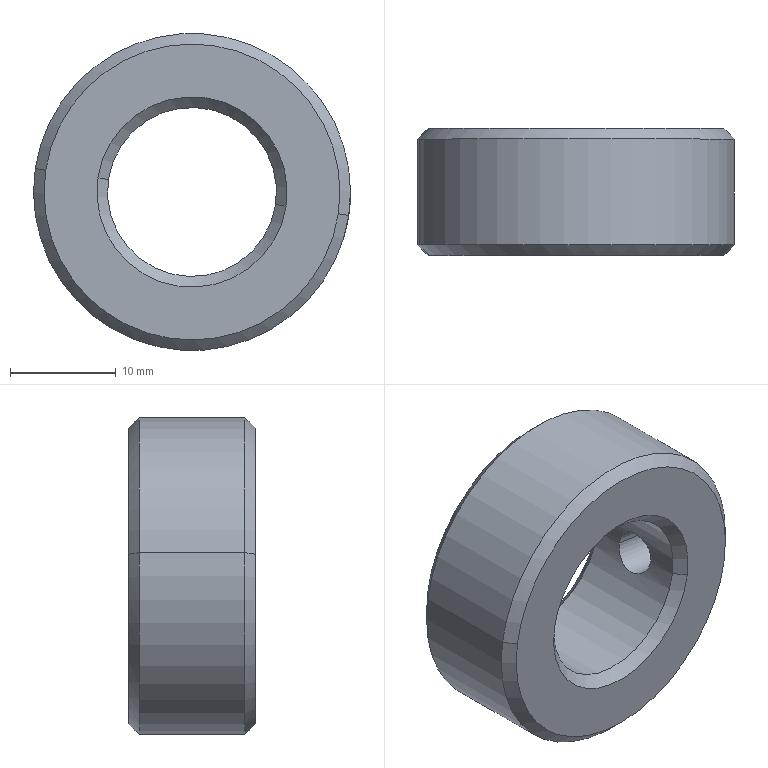Component | SolidWorks | LocatingRing-3 | 1 solid | 16 faces | box 30 x 12 x 30 mm | volume 5828 mm3 | cone 8 | cylinder 6 | plane 2 | commonest cylinder face diameters 30 x2 4.2 x2 16 x2
STEP:
#1=COLOUR_RGB('',0.7922,0.8196,0.9333);
#2=FILL_AREA_STYLE_COLOUR('',#1);
#3=FILL_AREA_STYLE('',(#2));
#4=SURFACE_STYLE_FILL_AREA(#3);
#5=SURFACE_SIDE_STYLE('',(#4));
#6=SURFACE_STYLE_USAGE(.BOTH.,#5);
#7=PRESENTATION_STYLE_ASSIGNMENT((#6));
#8=CARTESIAN_POINT('',(6.686,5.472,-5.796));
#9=VERTEX_POINT('',#8);
#10=CARTESIAN_POINT('',(5.518,5.472,-5.622));
#11=VERTEX_POINT('',#10);
#12=CARTESIAN_POINT('',(6.102,5.472,-5.709));
#13=DIRECTION('',(0.,-1.,0.));
#14=DIRECTION('',(0.9891,0.,-0.1473));
#15=AXIS2_PLACEMENT_3D('',#12,#13,#14);
#16=CIRCLE('',#15,0.5906);
#17=EDGE_CURVE('',#9,#11,#16,.T.);
#18=ORIENTED_EDGE('',*,*,#17,.T.);
#19=CARTESIAN_POINT('',(5.518,5.079,-5.622));
#20=VERTEX_POINT('',#19);
#21=CARTESIAN_POINT('',(5.518,5.512,-5.622));
#22=DIRECTION('',(0.,-1.,0.));
#23=VECTOR('',#22,39.37);
#24=LINE('',#21,#23);
#25=EDGE_CURVE('',#11,#20,#24,.T.);
#26=ORIENTED_EDGE('',*,*,#25,.T.);
#27=CARTESIAN_POINT('',(6.686,5.079,-5.796));
#28=VERTEX_POINT('',#27);
#29=CARTESIAN_POINT('',(6.102,5.079,-5.709));
#30=DIRECTION('',(-0.,1.,-0.));
#31=DIRECTION('',(0.9891,0.,-0.1473));
#32=AXIS2_PLACEMENT_3D('',#29,#30,#31);
#33=CIRCLE('',#32,0.5906);
#34=EDGE_CURVE('',#20,#28,#33,.T.);
#35=ORIENTED_EDGE('',*,*,#34,.T.);
#36=CARTESIAN_POINT('',(6.686,5.193,-5.796));
#37=VERTEX_POINT('',#36);
#38=CARTESIAN_POINT('',(6.686,5.512,-5.796));
#39=DIRECTION('',(0.,-1.,0.));
#40=VECTOR('',#39,39.37);
#41=LINE('',#38,#40);
#42=EDGE_CURVE('',#37,#28,#41,.T.);
#43=ORIENTED_EDGE('',*,*,#42,.F.);
#44=CARTESIAN_POINT('',(6.686,5.358,-5.796));
#45=VERTEX_POINT('',#44);
#46=CARTESIAN_POINT('',(6.686,5.193,-5.796));
#47=CARTESIAN_POINT('',(6.687,5.193,-5.79));
#48=CARTESIAN_POINT('',(6.688,5.193,-5.785));
#49=CARTESIAN_POINT('',(6.689,5.196,-5.774));
#50=CARTESIAN_POINT('',(6.69,5.197,-5.769));
#51=CARTESIAN_POINT('',(6.691,5.201,-5.759));
#52=CARTESIAN_POINT('',(6.691,5.204,-5.754));
#53=CARTESIAN_POINT('',(6.692,5.21,-5.745));
#54=CARTESIAN_POINT('',(6.692,5.213,-5.741));
#55=CARTESIAN_POINT('',(6.693,5.225,-5.73));
#56=CARTESIAN_POINT('',(6.693,5.234,-5.724));
#57=CARTESIAN_POINT('',(6.693,5.254,-5.715));
#58=CARTESIAN_POINT('',(6.693,5.265,-5.713));
#59=CARTESIAN_POINT('',(6.693,5.281,-5.713));
#60=CARTESIAN_POINT('',(6.693,5.286,-5.714));
#61=CARTESIAN_POINT('',(6.693,5.297,-5.716));
#62=CARTESIAN_POINT('',(6.693,5.302,-5.717));
#63=CARTESIAN_POINT('',(6.693,5.312,-5.721));
#64=CARTESIAN_POINT('',(6.693,5.317,-5.724));
#65=CARTESIAN_POINT('',(6.693,5.326,-5.73));
#66=CARTESIAN_POINT('',(6.692,5.33,-5.733));
#67=CARTESIAN_POINT('',(6.692,5.338,-5.741));
#68=CARTESIAN_POINT('',(6.692,5.341,-5.745));
#69=CARTESIAN_POINT('',(6.691,5.347,-5.754));
#70=CARTESIAN_POINT('',(6.691,5.35,-5.759));
#71=CARTESIAN_POINT('',(6.69,5.354,-5.769));
#72=CARTESIAN_POINT('',(6.689,5.356,-5.774));
#73=CARTESIAN_POINT('',(6.688,5.358,-5.785));
#74=CARTESIAN_POINT('',(6.687,5.358,-5.79));
#75=CARTESIAN_POINT('',(6.686,5.358,-5.796));
#76=B_SPLINE_CURVE_WITH_KNOTS('',3,(#46,#47,#48,#49,#50,#51,#52,#53,#54,#55,#56,#57,#58,#59,#60,#61,#62,#63,#64,#65,#66,#67,#68,#69,#70,#71,#72,#73,#74,#75),.UNSPECIFIED.,.F.,.F.,(4,2,2,2,2,2,2,2,2,2,2,2,2,2,4),(0.006572,0.006983,0.007394,0.007804,0.008215,0.009037,0.009858,0.01027,0.01068,0.01109,0.0115,0.01191,0.01232,0.01273,0.01314),.UNSPECIFIED.);
#77=EDGE_CURVE('',#37,#45,#76,.T.);
#78=ORIENTED_EDGE('',*,*,#77,.T.);
#79=CARTESIAN_POINT('',(6.686,5.512,-5.796));
#80=DIRECTION('',(0.,-1.,0.));
#81=VECTOR('',#80,39.37);
#82=LINE('',#79,#81);
#83=EDGE_CURVE('',#9,#45,#82,.T.);
#84=ORIENTED_EDGE('',*,*,#83,.F.);
#85=EDGE_LOOP('',(#18,#26,#35,#43,#78,#84));
#86=FACE_OUTER_BOUND('',#85,.T.);
#87=CARTESIAN_POINT('',(6.102,5.512,-5.709));
#88=DIRECTION('',(0.,-1.,0.));
#89=DIRECTION('',(0.9891,0.,-0.1473));
#90=AXIS2_PLACEMENT_3D('',#87,#88,#89);
#91=CYLINDRICAL_SURFACE('',#90,0.5906);
#92=ADVANCED_FACE('',(#86),#91,.T.);
#93=CARTESIAN_POINT('',(5.557,5.039,-5.627));
#94=VERTEX_POINT('',#93);
#95=CARTESIAN_POINT('',(6.648,5.039,-5.79));
#96=VERTEX_POINT('',#95);
#97=CARTESIAN_POINT('',(6.102,5.039,-5.709));
#98=DIRECTION('',(-0.,1.,-0.));
#99=DIRECTION('',(-0.9891,0.,0.1473));
#100=AXIS2_PLACEMENT_3D('',#97,#98,#99);
#101=CIRCLE('',#100,0.5512);
#102=EDGE_CURVE('',#94,#96,#101,.T.);
#103=ORIENTED_EDGE('',*,*,#102,.T.);
#104=CARTESIAN_POINT('',(6.686,5.079,-5.796));
#105=DIRECTION('',(0.6994,0.7071,-0.1041));
#106=VECTOR('',#105,39.37);
#107=LINE('',#104,#106);
#108=EDGE_CURVE('',#96,#28,#107,.T.);
#109=ORIENTED_EDGE('',*,*,#108,.T.);
#110=ORIENTED_EDGE('',*,*,#34,.F.);
#111=CARTESIAN_POINT('',(5.518,5.079,-5.622));
#112=DIRECTION('',(-0.6994,0.7071,0.1041));
#113=VECTOR('',#112,39.37);
#114=LINE('',#111,#113);
#115=EDGE_CURVE('',#94,#20,#114,.T.);
#116=ORIENTED_EDGE('',*,*,#115,.F.);
#117=EDGE_LOOP('',(#103,#109,#110,#116));
#118=FACE_OUTER_BOUND('',#117,.T.);
#119=CARTESIAN_POINT('',(6.102,5.079,-5.709));
#120=DIRECTION('',(-0.,1.,-0.));
#121=DIRECTION('',(-0.9891,0.,0.1473));
#122=AXIS2_PLACEMENT_3D('',#119,#120,#121);
#123=CONICAL_SURFACE('',#122,0.5906,0.7854);
#124=ADVANCED_FACE('',(#118),#123,.T.);
#125=CARTESIAN_POINT('',(6.414,5.193,-5.755));
#126=VERTEX_POINT('',#125);
#127=CARTESIAN_POINT('',(6.414,5.358,-5.755));
#128=VERTEX_POINT('',#127);
#129=CARTESIAN_POINT('',(6.414,5.193,-5.755));
#130=CARTESIAN_POINT('',(6.413,5.193,-5.76));
#131=CARTESIAN_POINT('',(6.412,5.193,-5.766));
#132=CARTESIAN_POINT('',(6.41,5.196,-5.776));
#133=CARTESIAN_POINT('',(6.409,5.197,-5.781));
#134=CARTESIAN_POINT('',(6.406,5.201,-5.791));
#135=CARTESIAN_POINT('',(6.405,5.204,-5.796));
#136=CARTESIAN_POINT('',(6.402,5.21,-5.804));
#137=CARTESIAN_POINT('',(6.401,5.213,-5.808));
#138=CARTESIAN_POINT('',(6.397,5.225,-5.819));
#139=CARTESIAN_POINT('',(6.395,5.234,-5.825));
#140=CARTESIAN_POINT('',(6.393,5.249,-5.831));
#141=CARTESIAN_POINT('',(6.392,5.254,-5.833));
#142=CARTESIAN_POINT('',(6.391,5.265,-5.835));
#143=CARTESIAN_POINT('',(6.391,5.27,-5.835));
#144=CARTESIAN_POINT('',(6.391,5.281,-5.835));
#145=CARTESIAN_POINT('',(6.391,5.286,-5.835));
#146=CARTESIAN_POINT('',(6.392,5.297,-5.833));
#147=CARTESIAN_POINT('',(6.393,5.302,-5.831));
#148=CARTESIAN_POINT('',(6.395,5.317,-5.825));
#149=CARTESIAN_POINT('',(6.397,5.326,-5.819));
#150=CARTESIAN_POINT('',(6.401,5.338,-5.808));
#151=CARTESIAN_POINT('',(6.402,5.341,-5.804));
#152=CARTESIAN_POINT('',(6.405,5.347,-5.796));
#153=CARTESIAN_POINT('',(6.406,5.35,-5.791));
#154=CARTESIAN_POINT('',(6.409,5.354,-5.781));
#155=CARTESIAN_POINT('',(6.41,5.356,-5.776));
#156=CARTESIAN_POINT('',(6.412,5.358,-5.766));
#157=CARTESIAN_POINT('',(6.413,5.358,-5.76));
#158=CARTESIAN_POINT('',(6.414,5.358,-5.755));
#159=B_SPLINE_CURVE_WITH_KNOTS('',3,(#129,#130,#131,#132,#133,#134,#135,#136,#137,#138,#139,#140,#141,#142,#143,#144,#145,#146,#147,#148,#149,#150,#151,#152,#153,#154,#155,#156,#157,#158),.UNSPECIFIED.,.F.,.F.,(4,2,2,2,2,2,2,2,2,2,2,2,2,2,4),(0.,0.000412,0.0008241,0.001236,0.001648,0.002472,0.002884,0.003296,0.003708,0.00412,0.004944,0.005356,0.005768,0.00618,0.006592),.UNSPECIFIED.);
#160=EDGE_CURVE('',#126,#128,#159,.T.);
#161=ORIENTED_EDGE('',*,*,#160,.F.);
#162=CARTESIAN_POINT('',(6.686,5.193,-5.796));
#163=DIRECTION('',(0.9891,0.,-0.1473));
#164=VECTOR('',#163,39.37);
#165=LINE('',#162,#164);
#166=EDGE_CURVE('',#126,#37,#165,.T.);
#167=ORIENTED_EDGE('',*,*,#166,.T.);
#168=CARTESIAN_POINT('',(6.686,5.358,-5.796));
#169=CARTESIAN_POINT('',(6.686,5.358,-5.801));
#170=CARTESIAN_POINT('',(6.685,5.358,-5.806));
#171=CARTESIAN_POINT('',(6.683,5.356,-5.817));
#172=CARTESIAN_POINT('',(6.682,5.354,-5.822));
#173=CARTESIAN_POINT('',(6.68,5.35,-5.832));
#174=CARTESIAN_POINT('',(6.679,5.347,-5.836));
#175=CARTESIAN_POINT('',(6.677,5.341,-5.845));
#176=CARTESIAN_POINT('',(6.676,5.338,-5.849));
#177=CARTESIAN_POINT('',(6.673,5.326,-5.86));
#178=CARTESIAN_POINT('',(6.671,5.317,-5.866));
#179=CARTESIAN_POINT('',(6.669,5.297,-5.874));
#180=CARTESIAN_POINT('',(6.669,5.286,-5.877));
#181=CARTESIAN_POINT('',(6.669,5.27,-5.877));
#182=CARTESIAN_POINT('',(6.669,5.265,-5.876));
#183=CARTESIAN_POINT('',(6.669,5.254,-5.874));
#184=CARTESIAN_POINT('',(6.67,5.249,-5.872));
#185=CARTESIAN_POINT('',(6.671,5.239,-5.868));
#186=CARTESIAN_POINT('',(6.672,5.234,-5.866));
#187=CARTESIAN_POINT('',(6.673,5.225,-5.86));
#188=CARTESIAN_POINT('',(6.674,5.221,-5.857));
#189=CARTESIAN_POINT('',(6.676,5.213,-5.849));
#190=CARTESIAN_POINT('',(6.677,5.21,-5.845));
#191=CARTESIAN_POINT('',(6.679,5.204,-5.837));
#192=CARTESIAN_POINT('',(6.68,5.201,-5.832));
#193=CARTESIAN_POINT('',(6.682,5.197,-5.822));
#194=CARTESIAN_POINT('',(6.683,5.196,-5.817));
#195=CARTESIAN_POINT('',(6.685,5.193,-5.806));
#196=CARTESIAN_POINT('',(6.686,5.193,-5.801));
#197=CARTESIAN_POINT('',(6.686,5.193,-5.796));
#198=B_SPLINE_CURVE_WITH_KNOTS('',3,(#168,#169,#170,#171,#172,#173,#174,#175,#176,#177,#178,#179,#180,#181,#182,#183,#184,#185,#186,#187,#188,#189,#190,#191,#192,#193,#194,#195,#196,#197),.UNSPECIFIED.,.F.,.F.,(4,2,2,2,2,2,2,2,2,2,2,2,2,2,4),(0.,0.0004108,0.0008215,0.001232,0.001643,0.002465,0.003286,0.003697,0.004108,0.004518,0.004929,0.00534,0.005751,0.006161,0.006572),.UNSPECIFIED.);
#199=EDGE_CURVE('',#45,#37,#198,.T.);
#200=ORIENTED_EDGE('',*,*,#199,.F.);
#201=CARTESIAN_POINT('',(6.686,5.358,-5.796));
#202=DIRECTION('',(0.9891,0.,-0.1473));
#203=VECTOR('',#202,39.37);
#204=LINE('',#201,#203);
#205=EDGE_CURVE('',#128,#45,#204,.T.);
#206=ORIENTED_EDGE('',*,*,#205,.F.);
#207=EDGE_LOOP('',(#161,#167,#200,#206));
#208=FACE_OUTER_BOUND('',#207,.T.);
#209=CARTESIAN_POINT('',(6.686,5.276,-5.796));
#210=DIRECTION('',(0.9891,0.,-0.1473));
#211=DIRECTION('',(0.,1.,0.));
#212=AXIS2_PLACEMENT_3D('',#209,#210,#211);
#213=CYLINDRICAL_SURFACE('',#212,0.08268);
#214=ADVANCED_FACE('',(#208),#213,.F.);
#215=CARTESIAN_POINT('',(6.648,5.512,-5.79));
#216=VERTEX_POINT('',#215);
#217=CARTESIAN_POINT('',(5.557,5.512,-5.627));
#218=VERTEX_POINT('',#217);
#219=CARTESIAN_POINT('',(6.102,5.512,-5.709));
#220=DIRECTION('',(0.,-1.,0.));
#221=DIRECTION('',(0.9891,0.,-0.1473));
#222=AXIS2_PLACEMENT_3D('',#219,#220,#221);
#223=CIRCLE('',#222,0.5512);
#224=EDGE_CURVE('',#216,#218,#223,.T.);
#225=ORIENTED_EDGE('',*,*,#224,.T.);
#226=CARTESIAN_POINT('',(5.518,5.472,-5.622));
#227=DIRECTION('',(-0.6994,-0.7071,0.1041));
#228=VECTOR('',#227,39.37);
#229=LINE('',#226,#228);
#230=EDGE_CURVE('',#218,#11,#229,.T.);
#231=ORIENTED_EDGE('',*,*,#230,.T.);
#232=ORIENTED_EDGE('',*,*,#17,.F.);
#233=CARTESIAN_POINT('',(6.686,5.472,-5.796));
#234=DIRECTION('',(0.6994,-0.7071,-0.1041));
#235=VECTOR('',#234,39.37);
#236=LINE('',#233,#235);
#237=EDGE_CURVE('',#216,#9,#236,.T.);
#238=ORIENTED_EDGE('',*,*,#237,.F.);
#239=EDGE_LOOP('',(#225,#231,#232,#238));
#240=FACE_OUTER_BOUND('',#239,.T.);
#241=CARTESIAN_POINT('',(6.102,5.472,-5.709));
#242=DIRECTION('',(0.,-1.,0.));
#243=DIRECTION('',(0.9891,0.,-0.1473));
#244=AXIS2_PLACEMENT_3D('',#241,#242,#243);
#245=CONICAL_SURFACE('',#244,0.5906,0.7854);
#246=ADVANCED_FACE('',(#240),#245,.T.);
#247=CARTESIAN_POINT('',(6.414,5.079,-5.755));
#248=VERTEX_POINT('',#247);
#249=CARTESIAN_POINT('',(5.791,5.079,-5.662));
#250=VERTEX_POINT('',#249);
#251=CARTESIAN_POINT('',(6.102,5.079,-5.709));
#252=DIRECTION('',(-0.,1.,-0.));
#253=DIRECTION('',(-0.9891,0.,0.1473));
#254=AXIS2_PLACEMENT_3D('',#251,#252,#253);
#255=CIRCLE('',#254,0.315);
#256=EDGE_CURVE('',#248,#250,#255,.T.);
#257=ORIENTED_EDGE('',*,*,#256,.F.);
#258=CARTESIAN_POINT('',(6.414,5.039,-5.755));
#259=DIRECTION('',(-0.,1.,-0.));
#260=VECTOR('',#259,39.37);
#261=LINE('',#258,#260);
#262=EDGE_CURVE('',#248,#126,#261,.T.);
#263=ORIENTED_EDGE('',*,*,#262,.T.);
#264=ORIENTED_EDGE('',*,*,#160,.T.);
#265=CARTESIAN_POINT('',(6.414,5.472,-5.755));
#266=VERTEX_POINT('',#265);
#267=CARTESIAN_POINT('',(6.414,5.039,-5.755));
#268=DIRECTION('',(-0.,1.,-0.));
#269=VECTOR('',#268,39.37);
#270=LINE('',#267,#269);
#271=EDGE_CURVE('',#128,#266,#270,.T.);
#272=ORIENTED_EDGE('',*,*,#271,.T.);
#273=CARTESIAN_POINT('',(5.791,5.472,-5.662));
#274=VERTEX_POINT('',#273);
#275=CARTESIAN_POINT('',(6.102,5.472,-5.709));
#276=DIRECTION('',(0.,-1.,0.));
#277=DIRECTION('',(-0.9891,0.,0.1473));
#278=AXIS2_PLACEMENT_3D('',#275,#276,#277);
#279=CIRCLE('',#278,0.315);
#280=EDGE_CURVE('',#274,#266,#279,.T.);
#281=ORIENTED_EDGE('',*,*,#280,.F.);
#282=CARTESIAN_POINT('',(5.791,5.039,-5.662));
#283=DIRECTION('',(-0.,1.,-0.));
#284=VECTOR('',#283,39.37);
#285=LINE('',#282,#284);
#286=EDGE_CURVE('',#250,#274,#285,.T.);
#287=ORIENTED_EDGE('',*,*,#286,.F.);
#288=EDGE_LOOP('',(#257,#263,#264,#272,#281,#287));
#289=FACE_OUTER_BOUND('',#288,.T.);
#290=CARTESIAN_POINT('',(6.102,5.039,-5.709));
#291=DIRECTION('',(-0.,1.,-0.));
#292=DIRECTION('',(-0.9891,0.,0.1473));
#293=AXIS2_PLACEMENT_3D('',#290,#291,#292);
#294=CYLINDRICAL_SURFACE('',#293,0.315);
#295=ADVANCED_FACE('',(#289),#294,.F.);
#296=ORIENTED_EDGE('',*,*,#256,.T.);
#297=CARTESIAN_POINT('',(5.752,5.039,-5.656));
#298=VERTEX_POINT('',#297);
#299=CARTESIAN_POINT('',(5.752,5.039,-5.656));
#300=DIRECTION('',(-0.6994,-0.7071,0.1041));
#301=VECTOR('',#300,39.37);
#302=LINE('',#299,#301);
#303=EDGE_CURVE('',#250,#298,#302,.T.);
#304=ORIENTED_EDGE('',*,*,#303,.T.);
#305=CARTESIAN_POINT('',(6.453,5.039,-5.761));
#306=VERTEX_POINT('',#305);
#307=CARTESIAN_POINT('',(6.102,5.039,-5.709));
#308=DIRECTION('',(0.,-1.,0.));
#309=DIRECTION('',(0.9891,0.,-0.1473));
#310=AXIS2_PLACEMENT_3D('',#307,#308,#309);
#311=CIRCLE('',#310,0.3543);
#312=EDGE_CURVE('',#298,#306,#311,.T.);
#313=ORIENTED_EDGE('',*,*,#312,.T.);
#314=CARTESIAN_POINT('',(6.453,5.039,-5.761));
#315=DIRECTION('',(0.6994,-0.7071,-0.1041));
#316=VECTOR('',#315,39.37);
#317=LINE('',#314,#316);
#318=EDGE_CURVE('',#248,#306,#317,.T.);
#319=ORIENTED_EDGE('',*,*,#318,.F.);
#320=EDGE_LOOP('',(#296,#304,#313,#319));
#321=FACE_OUTER_BOUND('',#320,.T.);
#322=CARTESIAN_POINT('',(6.102,5.039,-5.709));
#323=DIRECTION('',(0.,-1.,0.));
#324=DIRECTION('',(0.9891,0.,-0.1473));
#325=AXIS2_PLACEMENT_3D('',#322,#323,#324);
#326=CONICAL_SURFACE('',#325,0.3543,0.7854);
#327=ADVANCED_FACE('',(#321),#326,.F.);
#328=ORIENTED_EDGE('',*,*,#280,.T.);
#329=CARTESIAN_POINT('',(6.453,5.512,-5.761));
#330=VERTEX_POINT('',#329);
#331=CARTESIAN_POINT('',(6.453,5.512,-5.761));
#332=DIRECTION('',(0.6994,0.7071,-0.1041));
#333=VECTOR('',#332,39.37);
#334=LINE('',#331,#333);
#335=EDGE_CURVE('',#266,#330,#334,.T.);
#336=ORIENTED_EDGE('',*,*,#335,.T.);
#337=CARTESIAN_POINT('',(5.752,5.512,-5.656));
#338=VERTEX_POINT('',#337);
#339=CARTESIAN_POINT('',(6.102,5.512,-5.709));
#340=DIRECTION('',(0.,-1.,0.));
#341=DIRECTION('',(-0.9891,0.,0.1473));
#342=AXIS2_PLACEMENT_3D('',#339,#340,#341);
#343=CIRCLE('',#342,0.3543);
#344=EDGE_CURVE('',#338,#330,#343,.T.);
#345=ORIENTED_EDGE('',*,*,#344,.F.);
#346=CARTESIAN_POINT('',(5.752,5.512,-5.656));
#347=DIRECTION('',(-0.6994,0.7071,0.1041));
#348=VECTOR('',#347,39.37);
#349=LINE('',#346,#348);
#350=EDGE_CURVE('',#274,#338,#349,.T.);
#351=ORIENTED_EDGE('',*,*,#350,.F.);
#352=EDGE_LOOP('',(#328,#336,#345,#351));
#353=FACE_OUTER_BOUND('',#352,.T.);
#354=CARTESIAN_POINT('',(6.102,5.512,-5.709));
#355=DIRECTION('',(-0.,1.,-0.));
#356=DIRECTION('',(-0.9891,0.,0.1473));
#357=AXIS2_PLACEMENT_3D('',#354,#355,#356);
#358=CONICAL_SURFACE('',#357,0.3543,0.7854);
#359=ADVANCED_FACE('',(#353),#358,.F.);
#360=ORIENTED_EDGE('',*,*,#25,.F.);
#361=CARTESIAN_POINT('',(6.102,5.472,-5.709));
#362=DIRECTION('',(0.,-1.,0.));
#363=DIRECTION('',(0.9891,0.,-0.1473));
#364=AXIS2_PLACEMENT_3D('',#361,#362,#363);
#365=CIRCLE('',#364,0.5906);
#366=EDGE_CURVE('',#11,#9,#365,.T.);
#367=ORIENTED_EDGE('',*,*,#366,.T.);
#368=ORIENTED_EDGE('',*,*,#83,.T.);
#369=ORIENTED_EDGE('',*,*,#199,.T.);
#370=ORIENTED_EDGE('',*,*,#42,.T.);
#371=CARTESIAN_POINT('',(6.102,5.079,-5.709));
#372=DIRECTION('',(-0.,1.,-0.));
#373=DIRECTION('',(0.9891,0.,-0.1473));
#374=AXIS2_PLACEMENT_3D('',#371,#372,#373);
#375=CIRCLE('',#374,0.5906);
#376=EDGE_CURVE('',#28,#20,#375,.T.);
#377=ORIENTED_EDGE('',*,*,#376,.T.);
#378=EDGE_LOOP('',(#360,#367,#368,#369,#370,#377));
#379=FACE_OUTER_BOUND('',#378,.T.);
#380=CARTESIAN_POINT('',(6.102,5.512,-5.709));
#381=DIRECTION('',(0.,-1.,0.));
#382=DIRECTION('',(0.9891,0.,-0.1473));
#383=AXIS2_PLACEMENT_3D('',#380,#381,#382);
#384=CYLINDRICAL_SURFACE('',#383,0.5906);
#385=ADVANCED_FACE('',(#379),#384,.T.);
#386=ORIENTED_EDGE('',*,*,#108,.F.);
#387=CARTESIAN_POINT('',(6.102,5.039,-5.709));
#388=DIRECTION('',(-0.,1.,-0.));
#389=DIRECTION('',(-0.9891,0.,0.1473));
#390=AXIS2_PLACEMENT_3D('',#387,#388,#389);
#391=CIRCLE('',#390,0.5512);
#392=EDGE_CURVE('',#96,#94,#391,.T.);
#393=ORIENTED_EDGE('',*,*,#392,.T.);
#394=ORIENTED_EDGE('',*,*,#115,.T.);
#395=ORIENTED_EDGE('',*,*,#376,.F.);
#396=EDGE_LOOP('',(#386,#393,#394,#395));
#397=FACE_OUTER_BOUND('',#396,.T.);
#398=CARTESIAN_POINT('',(6.102,5.079,-5.709));
#399=DIRECTION('',(-0.,1.,-0.));
#400=DIRECTION('',(-0.9891,0.,0.1473));
#401=AXIS2_PLACEMENT_3D('',#398,#399,#400);
#402=CONICAL_SURFACE('',#401,0.5906,0.7854);
#403=ADVANCED_FACE('',(#397),#402,.T.);
#404=ORIENTED_EDGE('',*,*,#166,.F.);
#405=CARTESIAN_POINT('',(6.414,5.358,-5.755));
#406=CARTESIAN_POINT('',(6.415,5.358,-5.75));
#407=CARTESIAN_POINT('',(6.415,5.358,-5.744));
#408=CARTESIAN_POINT('',(6.416,5.356,-5.734));
#409=CARTESIAN_POINT('',(6.417,5.354,-5.728));
#410=CARTESIAN_POINT('',(6.417,5.35,-5.718));
#411=CARTESIAN_POINT('',(6.417,5.347,-5.714));
#412=CARTESIAN_POINT('',(6.417,5.341,-5.705));
#413=CARTESIAN_POINT('',(6.417,5.338,-5.7));
#414=CARTESIAN_POINT('',(6.417,5.326,-5.689));
#415=CARTESIAN_POINT('',(6.416,5.317,-5.682));
#416=CARTESIAN_POINT('',(6.416,5.302,-5.676));
#417=CARTESIAN_POINT('',(6.415,5.297,-5.674));
#418=CARTESIAN_POINT('',(6.415,5.286,-5.672));
#419=CARTESIAN_POINT('',(6.415,5.281,-5.672));
#420=CARTESIAN_POINT('',(6.415,5.27,-5.672));
#421=CARTESIAN_POINT('',(6.415,5.265,-5.672));
#422=CARTESIAN_POINT('',(6.415,5.254,-5.674));
#423=CARTESIAN_POINT('',(6.416,5.249,-5.676));
#424=CARTESIAN_POINT('',(6.416,5.234,-5.682));
#425=CARTESIAN_POINT('',(6.417,5.225,-5.689));
#426=CARTESIAN_POINT('',(6.417,5.213,-5.7));
#427=CARTESIAN_POINT('',(6.417,5.21,-5.704));
#428=CARTESIAN_POINT('',(6.417,5.204,-5.714));
#429=CARTESIAN_POINT('',(6.417,5.201,-5.718));
#430=CARTESIAN_POINT('',(6.417,5.197,-5.728));
#431=CARTESIAN_POINT('',(6.416,5.196,-5.734));
#432=CARTESIAN_POINT('',(6.415,5.193,-5.744));
#433=CARTESIAN_POINT('',(6.415,5.193,-5.75));
#434=CARTESIAN_POINT('',(6.414,5.193,-5.755));
#435=B_SPLINE_CURVE_WITH_KNOTS('',3,(#405,#406,#407,#408,#409,#410,#411,#412,#413,#414,#415,#416,#417,#418,#419,#420,#421,#422,#423,#424,#425,#426,#427,#428,#429,#430,#431,#432,#433,#434),.UNSPECIFIED.,.F.,.F.,(4,2,2,2,2,2,2,2,2,2,2,2,2,2,4),(0.006592,0.007004,0.007417,0.007829,0.008241,0.009065,0.009477,0.009889,0.0103,0.01071,0.01154,0.01195,0.01236,0.01277,0.01318),.UNSPECIFIED.);
#436=EDGE_CURVE('',#128,#126,#435,.T.);
#437=ORIENTED_EDGE('',*,*,#436,.F.);
#438=ORIENTED_EDGE('',*,*,#205,.T.);
#439=ORIENTED_EDGE('',*,*,#77,.F.);
#440=EDGE_LOOP('',(#404,#437,#438,#439));
#441=FACE_OUTER_BOUND('',#440,.T.);
#442=CARTESIAN_POINT('',(6.686,5.276,-5.796));
#443=DIRECTION('',(0.9891,0.,-0.1473));
#444=DIRECTION('',(0.,1.,0.));
#445=AXIS2_PLACEMENT_3D('',#442,#443,#444);
#446=CYLINDRICAL_SURFACE('',#445,0.08268);
#447=ADVANCED_FACE('',(#441),#446,.F.);
#448=ORIENTED_EDGE('',*,*,#230,.F.);
#449=CARTESIAN_POINT('',(6.102,5.512,-5.709));
#450=DIRECTION('',(0.,-1.,0.));
#451=DIRECTION('',(0.9891,0.,-0.1473));
#452=AXIS2_PLACEMENT_3D('',#449,#450,#451);
#453=CIRCLE('',#452,0.5512);
#454=EDGE_CURVE('',#218,#216,#453,.T.);
#455=ORIENTED_EDGE('',*,*,#454,.T.);
#456=ORIENTED_EDGE('',*,*,#237,.T.);
#457=ORIENTED_EDGE('',*,*,#366,.F.);
#458=EDGE_LOOP('',(#448,#455,#456,#457));
#459=FACE_OUTER_BOUND('',#458,.T.);
#460=CARTESIAN_POINT('',(6.102,5.472,-5.709));
#461=DIRECTION('',(0.,-1.,0.));
#462=DIRECTION('',(0.9891,0.,-0.1473));
#463=AXIS2_PLACEMENT_3D('',#460,#461,#462);
#464=CONICAL_SURFACE('',#463,0.5906,0.7854);
#465=ADVANCED_FACE('',(#459),#464,.T.);
#466=CARTESIAN_POINT('',(6.102,5.039,-5.709));
#467=DIRECTION('',(0.,-1.,0.));
#468=DIRECTION('',(0.9891,0.,-0.1473));
#469=AXIS2_PLACEMENT_3D('',#466,#467,#468);
#470=CIRCLE('',#469,0.3543);
#471=EDGE_CURVE('',#306,#298,#470,.T.);
#472=ORIENTED_EDGE('',*,*,#471,.F.);
#473=ORIENTED_EDGE('',*,*,#312,.F.);
#474=EDGE_LOOP('',(#472,#473));
#475=FACE_BOUND('',#474,.T.);
#476=ORIENTED_EDGE('',*,*,#102,.F.);
#477=ORIENTED_EDGE('',*,*,#392,.F.);
#478=EDGE_LOOP('',(#476,#477));
#479=FACE_OUTER_BOUND('',#478,.T.);
#480=CARTESIAN_POINT('',(6.102,5.039,-5.709));
#481=DIRECTION('',(-0.,1.,-0.));
#482=DIRECTION('',(-0.9891,-0.,0.1473));
#483=AXIS2_PLACEMENT_3D('',#480,#481,#482);
#484=PLANE('',#483);
#485=ADVANCED_FACE('',(#475,#479),#484,.F.);
#486=ORIENTED_EDGE('',*,*,#262,.F.);
#487=CARTESIAN_POINT('',(6.102,5.079,-5.709));
#488=DIRECTION('',(-0.,1.,-0.));
#489=DIRECTION('',(-0.9891,0.,0.1473));
#490=AXIS2_PLACEMENT_3D('',#487,#488,#489);
#491=CIRCLE('',#490,0.315);
#492=EDGE_CURVE('',#250,#248,#491,.T.);
#493=ORIENTED_EDGE('',*,*,#492,.F.);
#494=ORIENTED_EDGE('',*,*,#286,.T.);
#495=CARTESIAN_POINT('',(6.102,5.472,-5.709));
#496=DIRECTION('',(0.,-1.,0.));
#497=DIRECTION('',(-0.9891,0.,0.1473));
#498=AXIS2_PLACEMENT_3D('',#495,#496,#497);
#499=CIRCLE('',#498,0.315);
#500=EDGE_CURVE('',#266,#274,#499,.T.);
#501=ORIENTED_EDGE('',*,*,#500,.F.);
#502=ORIENTED_EDGE('',*,*,#271,.F.);
#503=ORIENTED_EDGE('',*,*,#436,.T.);
#504=EDGE_LOOP('',(#486,#493,#494,#501,#502,#503));
#505=FACE_OUTER_BOUND('',#504,.T.);
#506=CARTESIAN_POINT('',(6.102,5.039,-5.709));
#507=DIRECTION('',(-0.,1.,-0.));
#508=DIRECTION('',(-0.9891,0.,0.1473));
#509=AXIS2_PLACEMENT_3D('',#506,#507,#508);
#510=CYLINDRICAL_SURFACE('',#509,0.315);
#511=ADVANCED_FACE('',(#505),#510,.F.);
#512=ORIENTED_EDGE('',*,*,#344,.T.);
#513=CARTESIAN_POINT('',(6.102,5.512,-5.709));
#514=DIRECTION('',(0.,-1.,0.));
#515=DIRECTION('',(-0.9891,0.,0.1473));
#516=AXIS2_PLACEMENT_3D('',#513,#514,#515);
#517=CIRCLE('',#516,0.3543);
#518=EDGE_CURVE('',#330,#338,#517,.T.);
#519=ORIENTED_EDGE('',*,*,#518,.T.);
#520=EDGE_LOOP('',(#512,#519));
#521=FACE_BOUND('',#520,.T.);
#522=ORIENTED_EDGE('',*,*,#224,.F.);
#523=ORIENTED_EDGE('',*,*,#454,.F.);
#524=EDGE_LOOP('',(#522,#523));
#525=FACE_OUTER_BOUND('',#524,.T.);
#526=CARTESIAN_POINT('',(6.102,5.512,-5.709));
#527=DIRECTION('',(-0.,1.,-0.));
#528=DIRECTION('',(-0.9891,-0.,0.1473));
#529=AXIS2_PLACEMENT_3D('',#526,#527,#528);
#530=PLANE('',#529);
#531=ADVANCED_FACE('',(#521,#525),#530,.T.);
#532=ORIENTED_EDGE('',*,*,#303,.F.);
#533=ORIENTED_EDGE('',*,*,#492,.T.);
#534=ORIENTED_EDGE('',*,*,#318,.T.);
#535=ORIENTED_EDGE('',*,*,#471,.T.);
#536=EDGE_LOOP('',(#532,#533,#534,#535));
#537=FACE_OUTER_BOUND('',#536,.T.);
#538=CARTESIAN_POINT('',(6.102,5.039,-5.709));
#539=DIRECTION('',(0.,-1.,0.));
#540=DIRECTION('',(0.9891,0.,-0.1473));
#541=AXIS2_PLACEMENT_3D('',#538,#539,#540);
#542=CONICAL_SURFACE('',#541,0.3543,0.7854);
#543=ADVANCED_FACE('',(#537),#542,.F.);
#544=ORIENTED_EDGE('',*,*,#335,.F.);
#545=ORIENTED_EDGE('',*,*,#500,.T.);
#546=ORIENTED_EDGE('',*,*,#350,.T.);
#547=ORIENTED_EDGE('',*,*,#518,.F.);
#548=EDGE_LOOP('',(#544,#545,#546,#547));
#549=FACE_OUTER_BOUND('',#548,.T.);
#550=CARTESIAN_POINT('',(6.102,5.512,-5.709));
#551=DIRECTION('',(-0.,1.,-0.));
#552=DIRECTION('',(-0.9891,0.,0.1473));
#553=AXIS2_PLACEMENT_3D('',#550,#551,#552);
#554=CONICAL_SURFACE('',#553,0.3543,0.7854);
#555=ADVANCED_FACE('',(#549),#554,.F.);
#556=CLOSED_SHELL('',(#92,#124,#214,#246,#295,#327,#359,#385,#403,#447,#465,#485,#511,#531,#543,#555));
#557=MANIFOLD_SOLID_BREP('',#556);
#558=STYLED_ITEM('',(#7),#557);
#559=PRESENTATION_LAYER_ASSIGNMENT('','',(#558));
#560=CARTESIAN_POINT('',(0.,0.,0.));
#561=DIRECTION('',(0.,0.,1.));
#562=DIRECTION('',(1.,0.,0.));
#563=AXIS2_PLACEMENT_3D('',#560,#561,#562);
#564=(LENGTH_UNIT()NAMED_UNIT(*)SI_UNIT($,.METRE.));
#565=LENGTH_MEASURE_WITH_UNIT(LENGTH_MEASURE(0.0254),#564);
#566=DIMENSIONAL_EXPONENTS(1.,0.,0.,0.,0.,0.,0.);
#567=(CONVERSION_BASED_UNIT('',#565)LENGTH_UNIT()NAMED_UNIT(#566));
#568=UNCERTAINTY_MEASURE_WITH_UNIT(LENGTH_MEASURE(0.00001),#567,'','');
#569=(NAMED_UNIT(*)PLANE_ANGLE_UNIT()SI_UNIT($,.RADIAN.));
#570=(NAMED_UNIT(*)SI_UNIT($,.STERADIAN.)SOLID_ANGLE_UNIT());
#571=(GEOMETRIC_REPRESENTATION_CONTEXT(3)GLOBAL_UNCERTAINTY_ASSIGNED_CONTEXT((#568))GLOBAL_UNIT_ASSIGNED_CONTEXT((#567,#569,#570))REPRESENTATION_CONTEXT('',''));
#572=ADVANCED_BREP_SHAPE_REPRESENTATION('',(#557,#563),#571);
#573=(LENGTH_UNIT()NAMED_UNIT(*)SI_UNIT($,.METRE.));
#574=LENGTH_MEASURE_WITH_UNIT(LENGTH_MEASURE(0.0254),#573);
#575=DIMENSIONAL_EXPONENTS(1.,0.,0.,0.,0.,0.,0.);
#576=(CONVERSION_BASED_UNIT('',#574)LENGTH_UNIT()NAMED_UNIT(#575));
#577=UNCERTAINTY_MEASURE_WITH_UNIT(LENGTH_MEASURE(0.00001),#576,'','');
#578=(NAMED_UNIT(*)PLANE_ANGLE_UNIT()SI_UNIT($,.RADIAN.));
#579=(NAMED_UNIT(*)SI_UNIT($,.STERADIAN.)SOLID_ANGLE_UNIT());
#580=(GEOMETRIC_REPRESENTATION_CONTEXT(3)GLOBAL_UNCERTAINTY_ASSIGNED_CONTEXT((#577))GLOBAL_UNIT_ASSIGNED_CONTEXT((#576,#578,#579))REPRESENTATION_CONTEXT('',''));
#581=MECHANICAL_DESIGN_GEOMETRIC_PRESENTATION_REPRESENTATION('',(#558),#580);